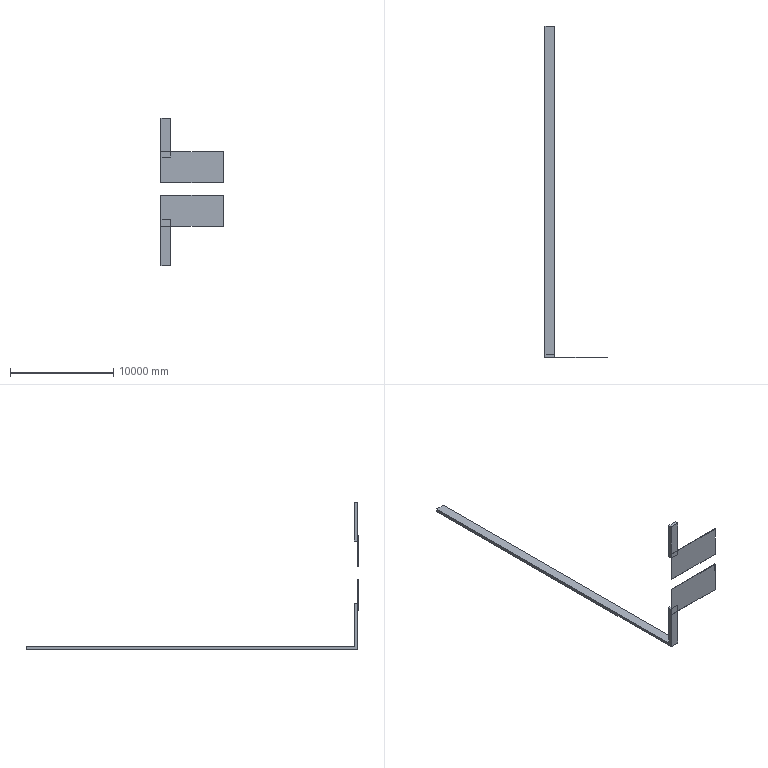Component | SolidWorks | Wall-1 | 4 solids | 26 faces | box 6000 x 32121.42 x 14227.61 mm | volume 12599737425 mm3 | plane 26
build123d program:
from build123d import *

# Parameters (mm, degrees)
BOSS_EXTRUDE1_DEPTH   = 900
SKETCH2_W             = 1916.372
SKETCH2_H             = 6000
CUT_EXTRUDE2_DEPTH    = 38704.356
SKETCH3_W             = 6000
SKETCH3_H             = 3000
BOSS_EXTRUDE2_DEPTH   = 50
BOSS_EXTRUDE2_2_DEPTH = 50


with BuildPart() as part:
    # Sketch1 → Boss-Extrude1 (new body)
    with BuildSketch(Plane.XY):
        Polygon((-3905.572, 13.034), (-35976.99, 13.034), (-35976.99, 313.034), (-35976.99, 14240.643), (-35676.99, 14240.643), (-35676.99, 313.034), (-3905.572, 313.034), align=None)
    extrude(amount=BOSS_EXTRUDE1_DEPTH)

    # Sketch2 → Cut-Extrude2 (cut, through all)
    with BuildSketch(Plane.XY.offset(900)):
        with Locations((-36116.386, 7513.034)):
            Rectangle(SKETCH2_W, SKETCH2_H)
    extrude(amount=-CUT_EXTRUDE2_DEPTH, mode=Mode.SUBTRACT)


with BuildPart() as cut_extrude2_piece_1:
    # of the separate pieces the step leaves, piece 1, a body of its own (cut_extrude2_pieces)
    add(part.part.solids().sort_by_distance((-3905.572, 13.034, 0))[0])


with BuildPart() as cut_extrude2_piece_2:
    # of the separate pieces the step leaves, piece 2, a body of its own (cut_extrude2_pieces)
    add(part.part.solids().sort_by_distance((-35976.99, 14240.643, 0))[0])


with BuildPart() as body_3:
    # Sketch3 → Boss-Extrude2 (new body)
    with BuildSketch(Plane.ZY.offset(35976.99)):
        with Locations((3000, 9513.138)):
            Rectangle(SKETCH3_W, SKETCH3_H)
    extrude(amount=BOSS_EXTRUDE2_DEPTH)


with BuildPart() as body_4:
    # Sketch3 → Boss-Extrude2 2 (new body)
    with BuildSketch(Plane.ZY.offset(35976.99)):
        with Locations((3000, 5329.239)):
            Rectangle(SKETCH3_W, SKETCH3_H)
    extrude(amount=BOSS_EXTRUDE2_2_DEPTH)


solid = Compound([cut_extrude2_piece_1.part, cut_extrude2_piece_2.part, body_3.part, body_4.part])

# Placed as in the assembly
solid = solid.moved(Location((-1730.074, 4663.226, -160.714), (90, 90, 0)))
STEP:
#1=CARTESIAN_POINT('',(-68.113,-1232.825,427.261));
#2=VERTEX_POINT('',#1);
#3=CARTESIAN_POINT('',(-68.113,-1232.825,309.151));
#4=VERTEX_POINT('',#3);
#5=CARTESIAN_POINT('',(-68.113,-1232.825,427.261));
#6=DIRECTION('',(-0.,-0.,-1.));
#7=VECTOR('',#6,39.37);
#8=LINE('',#5,#7);
#9=EDGE_CURVE('',#2,#4,#8,.T.);
#10=ORIENTED_EDGE('',*,*,#9,.T.);
#11=CARTESIAN_POINT('',(-68.113,-1234.794,309.151));
#12=VERTEX_POINT('',#11);
#13=CARTESIAN_POINT('',(-68.113,-1234.794,309.151));
#14=DIRECTION('',(0.,1.,-0.));
#15=VECTOR('',#14,39.37);
#16=LINE('',#13,#15);
#17=EDGE_CURVE('',#12,#4,#16,.T.);
#18=ORIENTED_EDGE('',*,*,#17,.F.);
#19=CARTESIAN_POINT('',(-68.113,-1234.794,427.261));
#20=VERTEX_POINT('',#19);
#21=CARTESIAN_POINT('',(-68.113,-1234.794,427.261));
#22=DIRECTION('',(-0.,-0.,-1.));
#23=VECTOR('',#22,39.37);
#24=LINE('',#21,#23);
#25=EDGE_CURVE('',#20,#12,#24,.T.);
#26=ORIENTED_EDGE('',*,*,#25,.F.);
#27=CARTESIAN_POINT('',(-68.113,-1234.794,427.261));
#28=DIRECTION('',(0.,1.,-0.));
#29=VECTOR('',#28,39.37);
#30=LINE('',#27,#29);
#31=EDGE_CURVE('',#20,#2,#30,.T.);
#32=ORIENTED_EDGE('',*,*,#31,.T.);
#33=EDGE_LOOP('',(#10,#18,#26,#32));
#34=FACE_OUTER_BOUND('',#33,.T.);
#35=CARTESIAN_POINT('',(-68.113,-1234.794,427.261));
#36=DIRECTION('',(1.,-0.,-0.));
#37=DIRECTION('',(-0.,-0.,-1.));
#38=AXIS2_PLACEMENT_3D('',#35,#36,#37);
#39=PLANE('',#38);
#40=ADVANCED_FACE('',(#34),#39,.F.);
#41=CARTESIAN_POINT('',(168.107,-1232.825,309.151));
#42=VERTEX_POINT('',#41);
#43=CARTESIAN_POINT('',(-68.113,-1232.825,309.151));
#44=DIRECTION('',(1.,-0.,-0.));
#45=VECTOR('',#44,39.37);
#46=LINE('',#43,#45);
#47=EDGE_CURVE('',#4,#42,#46,.T.);
#48=ORIENTED_EDGE('',*,*,#47,.T.);
#49=CARTESIAN_POINT('',(168.107,-1234.794,309.151));
#50=VERTEX_POINT('',#49);
#51=CARTESIAN_POINT('',(168.107,-1234.794,309.151));
#52=DIRECTION('',(0.,1.,-0.));
#53=VECTOR('',#52,39.37);
#54=LINE('',#51,#53);
#55=EDGE_CURVE('',#50,#42,#54,.T.);
#56=ORIENTED_EDGE('',*,*,#55,.F.);
#57=CARTESIAN_POINT('',(-68.113,-1234.794,309.151));
#58=DIRECTION('',(1.,-0.,-0.));
#59=VECTOR('',#58,39.37);
#60=LINE('',#57,#59);
#61=EDGE_CURVE('',#12,#50,#60,.T.);
#62=ORIENTED_EDGE('',*,*,#61,.F.);
#63=ORIENTED_EDGE('',*,*,#17,.T.);
#64=EDGE_LOOP('',(#48,#56,#62,#63));
#65=FACE_OUTER_BOUND('',#64,.T.);
#66=CARTESIAN_POINT('',(-68.113,-1234.794,309.151));
#67=DIRECTION('',(0.,0.,1.));
#68=DIRECTION('',(1.,-0.,-0.));
#69=AXIS2_PLACEMENT_3D('',#66,#67,#68);
#70=PLANE('',#69);
#71=ADVANCED_FACE('',(#65),#70,.F.);
#72=CARTESIAN_POINT('',(168.107,-1232.825,427.261));
#73=VERTEX_POINT('',#72);
#74=CARTESIAN_POINT('',(168.107,-1232.825,427.261));
#75=DIRECTION('',(0.,0.,1.));
#76=VECTOR('',#75,39.37);
#77=LINE('',#74,#76);
#78=EDGE_CURVE('',#42,#73,#77,.T.);
#79=ORIENTED_EDGE('',*,*,#78,.T.);
#80=CARTESIAN_POINT('',(168.107,-1234.794,427.261));
#81=VERTEX_POINT('',#80);
#82=CARTESIAN_POINT('',(168.107,-1234.794,427.261));
#83=DIRECTION('',(0.,1.,-0.));
#84=VECTOR('',#83,39.37);
#85=LINE('',#82,#84);
#86=EDGE_CURVE('',#81,#73,#85,.T.);
#87=ORIENTED_EDGE('',*,*,#86,.F.);
#88=CARTESIAN_POINT('',(168.107,-1234.794,427.261));
#89=DIRECTION('',(0.,0.,1.));
#90=VECTOR('',#89,39.37);
#91=LINE('',#88,#90);
#92=EDGE_CURVE('',#50,#81,#91,.T.);
#93=ORIENTED_EDGE('',*,*,#92,.F.);
#94=ORIENTED_EDGE('',*,*,#55,.T.);
#95=EDGE_LOOP('',(#79,#87,#93,#94));
#96=FACE_OUTER_BOUND('',#95,.T.);
#97=CARTESIAN_POINT('',(168.107,-1234.794,427.261));
#98=DIRECTION('',(-1.,0.,0.));
#99=DIRECTION('',(-0.,-1.,0.));
#100=AXIS2_PLACEMENT_3D('',#97,#98,#99);
#101=PLANE('',#100);
#102=ADVANCED_FACE('',(#96),#101,.F.);
#103=CARTESIAN_POINT('',(-68.113,-1232.825,427.261));
#104=DIRECTION('',(-1.,0.,0.));
#105=VECTOR('',#104,39.37);
#106=LINE('',#103,#105);
#107=EDGE_CURVE('',#73,#2,#106,.T.);
#108=ORIENTED_EDGE('',*,*,#107,.T.);
#109=ORIENTED_EDGE('',*,*,#31,.F.);
#110=CARTESIAN_POINT('',(-68.113,-1234.794,427.261));
#111=DIRECTION('',(-1.,0.,0.));
#112=VECTOR('',#111,39.37);
#113=LINE('',#110,#112);
#114=EDGE_CURVE('',#81,#20,#113,.T.);
#115=ORIENTED_EDGE('',*,*,#114,.F.);
#116=ORIENTED_EDGE('',*,*,#86,.T.);
#117=EDGE_LOOP('',(#108,#109,#115,#116));
#118=FACE_OUTER_BOUND('',#117,.T.);
#119=CARTESIAN_POINT('',(-68.113,-1234.794,427.261));
#120=DIRECTION('',(-0.,-0.,-1.));
#121=DIRECTION('',(-1.,0.,0.));
#122=AXIS2_PLACEMENT_3D('',#119,#120,#121);
#123=PLANE('',#122);
#124=ADVANCED_FACE('',(#118),#123,.F.);
#125=ORIENTED_EDGE('',*,*,#25,.T.);
#126=ORIENTED_EDGE('',*,*,#61,.T.);
#127=ORIENTED_EDGE('',*,*,#92,.T.);
#128=ORIENTED_EDGE('',*,*,#114,.T.);
#129=EDGE_LOOP('',(#125,#126,#127,#128));
#130=FACE_OUTER_BOUND('',#129,.T.);
#131=CARTESIAN_POINT('',(-68.113,-1234.794,-6.327));
#132=DIRECTION('',(-0.,-1.,0.));
#133=DIRECTION('',(1.,-0.,-0.));
#134=AXIS2_PLACEMENT_3D('',#131,#132,#133);
#135=PLANE('',#134);
#136=ADVANCED_FACE('',(#130),#135,.T.);
#137=ORIENTED_EDGE('',*,*,#9,.F.);
#138=ORIENTED_EDGE('',*,*,#107,.F.);
#139=ORIENTED_EDGE('',*,*,#78,.F.);
#140=ORIENTED_EDGE('',*,*,#47,.F.);
#141=EDGE_LOOP('',(#137,#138,#139,#140));
#142=FACE_OUTER_BOUND('',#141,.T.);
#143=CARTESIAN_POINT('',(-68.113,-1232.825,-6.327));
#144=DIRECTION('',(-0.,-1.,0.));
#145=DIRECTION('',(1.,-0.,-0.));
#146=AXIS2_PLACEMENT_3D('',#143,#144,#145);
#147=PLANE('',#146);
#148=ADVANCED_FACE('',(#142),#147,.F.);
#149=CLOSED_SHELL('',(#40,#71,#102,#124,#136,#148));
#150=MANIFOLD_SOLID_BREP('',#149);
#151=CARTESIAN_POINT('',(-68.113,-1232.825,554.328));
#152=VERTEX_POINT('',#151);
#153=CARTESIAN_POINT('',(-68.113,-1221.014,554.328));
#154=VERTEX_POINT('',#153);
#155=CARTESIAN_POINT('',(-68.113,-1232.825,554.328));
#156=DIRECTION('',(0.,1.,-0.));
#157=VECTOR('',#156,39.37);
#158=LINE('',#155,#157);
#159=EDGE_CURVE('',#152,#154,#158,.T.);
#160=ORIENTED_EDGE('',*,*,#159,.F.);
#161=CARTESIAN_POINT('',(-32.68,-1232.825,554.328));
#162=VERTEX_POINT('',#161);
#163=CARTESIAN_POINT('',(-32.68,-1232.825,554.328));
#164=DIRECTION('',(-1.,0.,0.));
#165=VECTOR('',#164,39.37);
#166=LINE('',#163,#165);
#167=EDGE_CURVE('',#162,#152,#166,.T.);
#168=ORIENTED_EDGE('',*,*,#167,.F.);
#169=CARTESIAN_POINT('',(-32.68,-1221.014,554.328));
#170=VERTEX_POINT('',#169);
#171=CARTESIAN_POINT('',(-32.68,-1232.825,554.328));
#172=DIRECTION('',(0.,1.,-0.));
#173=VECTOR('',#172,39.37);
#174=LINE('',#171,#173);
#175=EDGE_CURVE('',#162,#170,#174,.T.);
#176=ORIENTED_EDGE('',*,*,#175,.T.);
#177=CARTESIAN_POINT('',(-32.68,-1221.014,554.328));
#178=DIRECTION('',(-1.,0.,0.));
#179=VECTOR('',#178,39.37);
#180=LINE('',#177,#179);
#181=EDGE_CURVE('',#170,#154,#180,.T.);
#182=ORIENTED_EDGE('',*,*,#181,.T.);
#183=EDGE_LOOP('',(#160,#168,#176,#182));
#184=FACE_OUTER_BOUND('',#183,.T.);
#185=CARTESIAN_POINT('',(-32.68,-1232.825,554.328));
#186=DIRECTION('',(0.,0.,1.));
#187=DIRECTION('',(1.,-0.,-0.));
#188=AXIS2_PLACEMENT_3D('',#185,#186,#187);
#189=PLANE('',#188);
#190=ADVANCED_FACE('',(#184),#189,.T.);
#191=CARTESIAN_POINT('',(-68.113,-1232.825,407.572));
#192=VERTEX_POINT('',#191);
#193=CARTESIAN_POINT('',(-68.113,-1221.014,407.572));
#194=VERTEX_POINT('',#193);
#195=CARTESIAN_POINT('',(-68.113,183.592,407.572));
#196=DIRECTION('',(0.,1.,-0.));
#197=VECTOR('',#196,39.37);
#198=LINE('',#195,#197);
#199=EDGE_CURVE('',#192,#194,#198,.T.);
#200=ORIENTED_EDGE('',*,*,#199,.F.);
#201=CARTESIAN_POINT('',(-68.113,-1232.825,5.997));
#202=DIRECTION('',(0.,0.,1.));
#203=VECTOR('',#202,39.37);
#204=LINE('',#201,#203);
#205=EDGE_CURVE('',#192,#152,#204,.T.);
#206=ORIENTED_EDGE('',*,*,#205,.T.);
#207=ORIENTED_EDGE('',*,*,#159,.T.);
#208=CARTESIAN_POINT('',(-68.113,-1221.014,5.997));
#209=DIRECTION('',(0.,0.,1.));
#210=VECTOR('',#209,39.37);
#211=LINE('',#208,#210);
#212=EDGE_CURVE('',#194,#154,#211,.T.);
#213=ORIENTED_EDGE('',*,*,#212,.F.);
#214=EDGE_LOOP('',(#200,#206,#207,#213));
#215=FACE_OUTER_BOUND('',#214,.T.);
#216=CARTESIAN_POINT('',(-68.113,183.592,-6.327));
#217=DIRECTION('',(-1.,0.,0.));
#218=DIRECTION('',(-0.,-1.,0.));
#219=AXIS2_PLACEMENT_3D('',#216,#217,#218);
#220=PLANE('',#219);
#221=ADVANCED_FACE('',(#215),#220,.T.);
#222=CARTESIAN_POINT('',(-32.68,-1232.825,407.572));
#223=VERTEX_POINT('',#222);
#224=CARTESIAN_POINT('',(-32.68,-1232.825,-5.814));
#225=DIRECTION('',(0.,0.,1.));
#226=VECTOR('',#225,39.37);
#227=LINE('',#224,#226);
#228=EDGE_CURVE('',#223,#162,#227,.T.);
#229=ORIENTED_EDGE('',*,*,#228,.F.);
#230=CARTESIAN_POINT('',(-32.68,-1221.014,407.572));
#231=VERTEX_POINT('',#230);
#232=CARTESIAN_POINT('',(-32.68,-1200.59,407.572));
#233=DIRECTION('',(-0.,-1.,0.));
#234=VECTOR('',#233,39.37);
#235=LINE('',#232,#234);
#236=EDGE_CURVE('',#231,#223,#235,.T.);
#237=ORIENTED_EDGE('',*,*,#236,.F.);
#238=CARTESIAN_POINT('',(-32.68,-1221.014,5.997));
#239=DIRECTION('',(0.,0.,1.));
#240=VECTOR('',#239,39.37);
#241=LINE('',#238,#240);
#242=EDGE_CURVE('',#231,#170,#241,.T.);
#243=ORIENTED_EDGE('',*,*,#242,.T.);
#244=ORIENTED_EDGE('',*,*,#175,.F.);
#245=EDGE_LOOP('',(#229,#237,#243,#244));
#246=FACE_OUTER_BOUND('',#245,.T.);
#247=CARTESIAN_POINT('',(-32.68,183.592,-6.327));
#248=DIRECTION('',(-1.,0.,0.));
#249=DIRECTION('',(-0.,-1.,0.));
#250=AXIS2_PLACEMENT_3D('',#247,#248,#249);
#251=PLANE('',#250);
#252=ADVANCED_FACE('',(#246),#251,.F.);
#253=CARTESIAN_POINT('',(-32.68,-1232.825,407.572));
#254=DIRECTION('',(-1.,0.,0.));
#255=VECTOR('',#254,39.37);
#256=LINE('',#253,#255);
#257=EDGE_CURVE('',#223,#192,#256,.T.);
#258=ORIENTED_EDGE('',*,*,#257,.F.);
#259=ORIENTED_EDGE('',*,*,#228,.T.);
#260=ORIENTED_EDGE('',*,*,#167,.T.);
#261=ORIENTED_EDGE('',*,*,#205,.F.);
#262=EDGE_LOOP('',(#258,#259,#260,#261));
#263=FACE_OUTER_BOUND('',#262,.T.);
#264=CARTESIAN_POINT('',(-32.68,-1232.825,5.997));
#265=DIRECTION('',(-0.,-1.,0.));
#266=DIRECTION('',(1.,-0.,-0.));
#267=AXIS2_PLACEMENT_3D('',#264,#265,#266);
#268=PLANE('',#267);
#269=ADVANCED_FACE('',(#263),#268,.T.);
#270=ORIENTED_EDGE('',*,*,#242,.F.);
#271=CARTESIAN_POINT('',(-32.68,-1221.014,407.572));
#272=DIRECTION('',(-1.,0.,0.));
#273=VECTOR('',#272,39.37);
#274=LINE('',#271,#273);
#275=EDGE_CURVE('',#231,#194,#274,.T.);
#276=ORIENTED_EDGE('',*,*,#275,.T.);
#277=ORIENTED_EDGE('',*,*,#212,.T.);
#278=ORIENTED_EDGE('',*,*,#181,.F.);
#279=EDGE_LOOP('',(#270,#276,#277,#278));
#280=FACE_OUTER_BOUND('',#279,.T.);
#281=CARTESIAN_POINT('',(-32.68,-1221.014,5.997));
#282=DIRECTION('',(-0.,-1.,0.));
#283=DIRECTION('',(1.,-0.,-0.));
#284=AXIS2_PLACEMENT_3D('',#281,#282,#283);
#285=PLANE('',#284);
#286=ADVANCED_FACE('',(#280),#285,.F.);
#287=ORIENTED_EDGE('',*,*,#236,.T.);
#288=ORIENTED_EDGE('',*,*,#257,.T.);
#289=ORIENTED_EDGE('',*,*,#199,.T.);
#290=ORIENTED_EDGE('',*,*,#275,.F.);
#291=EDGE_LOOP('',(#287,#288,#289,#290));
#292=FACE_OUTER_BOUND('',#291,.T.);
#293=CARTESIAN_POINT('',(-68.113,-1200.59,407.572));
#294=DIRECTION('',(0.,0.,1.));
#295=DIRECTION('',(1.,-0.,-0.));
#296=AXIS2_PLACEMENT_3D('',#293,#294,#295);
#297=PLANE('',#296);
#298=ADVANCED_FACE('',(#292),#297,.F.);
#299=CLOSED_SHELL('',(#190,#221,#252,#269,#286,#298));
#300=MANIFOLD_SOLID_BREP('',#299);
#301=CARTESIAN_POINT('',(-68.113,-1221.014,5.997));
#302=VERTEX_POINT('',#301);
#303=CARTESIAN_POINT('',(-68.113,-1221.014,171.351));
#304=VERTEX_POINT('',#303);
#305=CARTESIAN_POINT('',(-68.113,-1221.014,5.997));
#306=DIRECTION('',(0.,0.,1.));
#307=VECTOR('',#306,39.37);
#308=LINE('',#305,#307);
#309=EDGE_CURVE('',#302,#304,#308,.T.);
#310=ORIENTED_EDGE('',*,*,#309,.T.);
#311=CARTESIAN_POINT('',(-32.68,-1221.014,171.351));
#312=VERTEX_POINT('',#311);
#313=CARTESIAN_POINT('',(-32.68,-1221.014,171.351));
#314=DIRECTION('',(1.,-0.,-0.));
#315=VECTOR('',#314,39.37);
#316=LINE('',#313,#315);
#317=EDGE_CURVE('',#304,#312,#316,.T.);
#318=ORIENTED_EDGE('',*,*,#317,.T.);
#319=CARTESIAN_POINT('',(-32.68,-1221.014,5.997));
#320=VERTEX_POINT('',#319);
#321=CARTESIAN_POINT('',(-32.68,-1221.014,5.997));
#322=DIRECTION('',(0.,0.,1.));
#323=VECTOR('',#322,39.37);
#324=LINE('',#321,#323);
#325=EDGE_CURVE('',#320,#312,#324,.T.);
#326=ORIENTED_EDGE('',*,*,#325,.F.);
#327=CARTESIAN_POINT('',(-32.68,-1221.014,5.997));
#328=DIRECTION('',(-1.,0.,0.));
#329=VECTOR('',#328,39.37);
#330=LINE('',#327,#329);
#331=EDGE_CURVE('',#320,#302,#330,.T.);
#332=ORIENTED_EDGE('',*,*,#331,.T.);
#333=EDGE_LOOP('',(#310,#318,#326,#332));
#334=FACE_OUTER_BOUND('',#333,.T.);
#335=CARTESIAN_POINT('',(-32.68,-1221.014,5.997));
#336=DIRECTION('',(-0.,-1.,0.));
#337=DIRECTION('',(1.,-0.,-0.));
#338=AXIS2_PLACEMENT_3D('',#335,#336,#337);
#339=PLANE('',#338);
#340=ADVANCED_FACE('',(#334),#339,.F.);
#341=CARTESIAN_POINT('',(-68.113,-1232.825,171.351));
#342=VERTEX_POINT('',#341);
#343=CARTESIAN_POINT('',(-32.68,-1232.825,171.351));
#344=VERTEX_POINT('',#343);
#345=CARTESIAN_POINT('',(-32.68,-1232.825,171.351));
#346=DIRECTION('',(1.,-0.,-0.));
#347=VECTOR('',#346,39.37);
#348=LINE('',#345,#347);
#349=EDGE_CURVE('',#342,#344,#348,.T.);
#350=ORIENTED_EDGE('',*,*,#349,.F.);
#351=CARTESIAN_POINT('',(-68.113,-1232.825,-5.814));
#352=VERTEX_POINT('',#351);
#353=CARTESIAN_POINT('',(-68.113,-1232.825,5.997));
#354=DIRECTION('',(0.,0.,1.));
#355=VECTOR('',#354,39.37);
#356=LINE('',#353,#355);
#357=EDGE_CURVE('',#352,#342,#356,.T.);
#358=ORIENTED_EDGE('',*,*,#357,.F.);
#359=CARTESIAN_POINT('',(-32.68,-1232.825,-5.814));
#360=VERTEX_POINT('',#359);
#361=CARTESIAN_POINT('',(-32.68,-1232.825,-5.814));
#362=DIRECTION('',(-1.,0.,0.));
#363=VECTOR('',#362,39.37);
#364=LINE('',#361,#363);
#365=EDGE_CURVE('',#360,#352,#364,.T.);
#366=ORIENTED_EDGE('',*,*,#365,.F.);
#367=CARTESIAN_POINT('',(-32.68,-1232.825,-5.814));
#368=DIRECTION('',(0.,0.,1.));
#369=VECTOR('',#368,39.37);
#370=LINE('',#367,#369);
#371=EDGE_CURVE('',#360,#344,#370,.T.);
#372=ORIENTED_EDGE('',*,*,#371,.T.);
#373=EDGE_LOOP('',(#350,#358,#366,#372));
#374=FACE_OUTER_BOUND('',#373,.T.);
#375=CARTESIAN_POINT('',(-32.68,-1232.825,5.997));
#376=DIRECTION('',(-0.,-1.,0.));
#377=DIRECTION('',(1.,-0.,-0.));
#378=AXIS2_PLACEMENT_3D('',#375,#376,#377);
#379=PLANE('',#378);
#380=ADVANCED_FACE('',(#374),#379,.T.);
#381=ORIENTED_EDGE('',*,*,#325,.T.);
#382=CARTESIAN_POINT('',(-32.68,-1200.59,171.351));
#383=DIRECTION('',(0.,1.,-0.));
#384=VECTOR('',#383,39.37);
#385=LINE('',#382,#384);
#386=EDGE_CURVE('',#344,#312,#385,.T.);
#387=ORIENTED_EDGE('',*,*,#386,.F.);
#388=ORIENTED_EDGE('',*,*,#371,.F.);
#389=CARTESIAN_POINT('',(-32.68,29.829,-5.814));
#390=VERTEX_POINT('',#389);
#391=CARTESIAN_POINT('',(-32.68,29.829,-5.814));
#392=DIRECTION('',(-0.,-1.,0.));
#393=VECTOR('',#392,39.37);
#394=LINE('',#391,#393);
#395=EDGE_CURVE('',#390,#360,#394,.T.);
#396=ORIENTED_EDGE('',*,*,#395,.F.);
#397=CARTESIAN_POINT('',(-32.68,29.829,5.997));
#398=VERTEX_POINT('',#397);
#399=CARTESIAN_POINT('',(-32.68,29.829,-5.814));
#400=DIRECTION('',(0.,0.,1.));
#401=VECTOR('',#400,39.37);
#402=LINE('',#399,#401);
#403=EDGE_CURVE('',#390,#398,#402,.T.);
#404=ORIENTED_EDGE('',*,*,#403,.T.);
#405=CARTESIAN_POINT('',(-32.68,29.829,5.997));
#406=DIRECTION('',(-0.,-1.,0.));
#407=VECTOR('',#406,39.37);
#408=LINE('',#405,#407);
#409=EDGE_CURVE('',#398,#320,#408,.T.);
#410=ORIENTED_EDGE('',*,*,#409,.T.);
#411=EDGE_LOOP('',(#381,#387,#388,#396,#404,#410));
#412=FACE_OUTER_BOUND('',#411,.T.);
#413=CARTESIAN_POINT('',(-32.68,183.592,-6.327));
#414=DIRECTION('',(-1.,0.,0.));
#415=DIRECTION('',(-0.,-1.,0.));
#416=AXIS2_PLACEMENT_3D('',#413,#414,#415);
#417=PLANE('',#416);
#418=ADVANCED_FACE('',(#412),#417,.F.);
#419=CARTESIAN_POINT('',(-68.113,183.592,171.351));
#420=DIRECTION('',(-0.,-1.,0.));
#421=VECTOR('',#420,39.37);
#422=LINE('',#419,#421);
#423=EDGE_CURVE('',#304,#342,#422,.T.);
#424=ORIENTED_EDGE('',*,*,#423,.F.);
#425=ORIENTED_EDGE('',*,*,#309,.F.);
#426=CARTESIAN_POINT('',(-68.113,29.829,5.997));
#427=VERTEX_POINT('',#426);
#428=CARTESIAN_POINT('',(-68.113,29.829,5.997));
#429=DIRECTION('',(-0.,-1.,0.));
#430=VECTOR('',#429,39.37);
#431=LINE('',#428,#430);
#432=EDGE_CURVE('',#427,#302,#431,.T.);
#433=ORIENTED_EDGE('',*,*,#432,.F.);
#434=CARTESIAN_POINT('',(-68.113,29.829,-5.814));
#435=VERTEX_POINT('',#434);
#436=CARTESIAN_POINT('',(-68.113,29.829,-5.814));
#437=DIRECTION('',(0.,0.,1.));
#438=VECTOR('',#437,39.37);
#439=LINE('',#436,#438);
#440=EDGE_CURVE('',#435,#427,#439,.T.);
#441=ORIENTED_EDGE('',*,*,#440,.F.);
#442=CARTESIAN_POINT('',(-68.113,29.829,-5.814));
#443=DIRECTION('',(-0.,-1.,0.));
#444=VECTOR('',#443,39.37);
#445=LINE('',#442,#444);
#446=EDGE_CURVE('',#435,#352,#445,.T.);
#447=ORIENTED_EDGE('',*,*,#446,.T.);
#448=ORIENTED_EDGE('',*,*,#357,.T.);
#449=EDGE_LOOP('',(#424,#425,#433,#441,#447,#448));
#450=FACE_OUTER_BOUND('',#449,.T.);
#451=CARTESIAN_POINT('',(-68.113,183.592,-6.327));
#452=DIRECTION('',(-1.,0.,0.));
#453=DIRECTION('',(-0.,-1.,0.));
#454=AXIS2_PLACEMENT_3D('',#451,#452,#453);
#455=PLANE('',#454);
#456=ADVANCED_FACE('',(#450),#455,.T.);
#457=ORIENTED_EDGE('',*,*,#446,.F.);
#458=CARTESIAN_POINT('',(-32.68,29.829,-5.814));
#459=DIRECTION('',(-1.,0.,0.));
#460=VECTOR('',#459,39.37);
#461=LINE('',#458,#460);
#462=EDGE_CURVE('',#390,#435,#461,.T.);
#463=ORIENTED_EDGE('',*,*,#462,.F.);
#464=ORIENTED_EDGE('',*,*,#395,.T.);
#465=ORIENTED_EDGE('',*,*,#365,.T.);
#466=EDGE_LOOP('',(#457,#463,#464,#465));
#467=FACE_OUTER_BOUND('',#466,.T.);
#468=CARTESIAN_POINT('',(-32.68,29.829,-5.814));
#469=DIRECTION('',(-0.,-0.,-1.));
#470=DIRECTION('',(-1.,0.,0.));
#471=AXIS2_PLACEMENT_3D('',#468,#469,#470);
#472=PLANE('',#471);
#473=ADVANCED_FACE('',(#467),#472,.T.);
#474=ORIENTED_EDGE('',*,*,#440,.T.);
#475=CARTESIAN_POINT('',(-32.68,29.829,5.997));
#476=DIRECTION('',(-1.,0.,0.));
#477=VECTOR('',#476,39.37);
#478=LINE('',#475,#477);
#479=EDGE_CURVE('',#398,#427,#478,.T.);
#480=ORIENTED_EDGE('',*,*,#479,.F.);
#481=ORIENTED_EDGE('',*,*,#403,.F.);
#482=ORIENTED_EDGE('',*,*,#462,.T.);
#483=EDGE_LOOP('',(#474,#480,#481,#482));
#484=FACE_OUTER_BOUND('',#483,.T.);
#485=CARTESIAN_POINT('',(-32.68,29.829,-5.814));
#486=DIRECTION('',(-0.,-1.,0.));
#487=DIRECTION('',(1.,-0.,-0.));
#488=AXIS2_PLACEMENT_3D('',#485,#486,#487);
#489=PLANE('',#488);
#490=ADVANCED_FACE('',(#484),#489,.F.);
#491=ORIENTED_EDGE('',*,*,#432,.T.);
#492=ORIENTED_EDGE('',*,*,#331,.F.);
#493=ORIENTED_EDGE('',*,*,#409,.F.);
#494=ORIENTED_EDGE('',*,*,#479,.T.);
#495=EDGE_LOOP('',(#491,#492,#493,#494));
#496=FACE_OUTER_BOUND('',#495,.T.);
#497=CARTESIAN_POINT('',(-32.68,29.829,5.997));
#498=DIRECTION('',(-0.,-0.,-1.));
#499=DIRECTION('',(-1.,0.,0.));
#500=AXIS2_PLACEMENT_3D('',#497,#498,#499);
#501=PLANE('',#500);
#502=ADVANCED_FACE('',(#496),#501,.F.);
#503=ORIENTED_EDGE('',*,*,#423,.T.);
#504=ORIENTED_EDGE('',*,*,#349,.T.);
#505=ORIENTED_EDGE('',*,*,#386,.T.);
#506=ORIENTED_EDGE('',*,*,#317,.F.);
#507=EDGE_LOOP('',(#503,#504,#505,#506));
#508=FACE_OUTER_BOUND('',#507,.T.);
#509=CARTESIAN_POINT('',(-68.113,-1200.59,171.351));
#510=DIRECTION('',(-0.,-0.,-1.));
#511=DIRECTION('',(-1.,0.,0.));
#512=AXIS2_PLACEMENT_3D('',#509,#510,#511);
#513=PLANE('',#512);
#514=ADVANCED_FACE('',(#508),#513,.F.);
#515=CLOSED_SHELL('',(#340,#380,#418,#456,#473,#490,#502,#514));
#516=MANIFOLD_SOLID_BREP('',#515);
#517=CARTESIAN_POINT('',(-68.113,-1232.825,262.54));
#518=VERTEX_POINT('',#517);
#519=CARTESIAN_POINT('',(-68.113,-1232.825,144.43));
#520=VERTEX_POINT('',#519);
#521=CARTESIAN_POINT('',(-68.113,-1232.825,144.43));
#522=DIRECTION('',(-0.,-0.,-1.));
#523=VECTOR('',#522,39.37);
#524=LINE('',#521,#523);
#525=EDGE_CURVE('',#518,#520,#524,.T.);
#526=ORIENTED_EDGE('',*,*,#525,.T.);
#527=CARTESIAN_POINT('',(-68.113,-1234.794,144.43));
#528=VERTEX_POINT('',#527);
#529=CARTESIAN_POINT('',(-68.113,-1234.794,144.43));
#530=DIRECTION('',(0.,1.,-0.));
#531=VECTOR('',#530,39.37);
#532=LINE('',#529,#531);
#533=EDGE_CURVE('',#528,#520,#532,.T.);
#534=ORIENTED_EDGE('',*,*,#533,.F.);
#535=CARTESIAN_POINT('',(-68.113,-1234.794,262.54));
#536=VERTEX_POINT('',#535);
#537=CARTESIAN_POINT('',(-68.113,-1234.794,144.43));
#538=DIRECTION('',(-0.,-0.,-1.));
#539=VECTOR('',#538,39.37);
#540=LINE('',#537,#539);
#541=EDGE_CURVE('',#536,#528,#540,.T.);
#542=ORIENTED_EDGE('',*,*,#541,.F.);
#543=CARTESIAN_POINT('',(-68.113,-1234.794,262.54));
#544=DIRECTION('',(0.,1.,-0.));
#545=VECTOR('',#544,39.37);
#546=LINE('',#543,#545);
#547=EDGE_CURVE('',#536,#518,#546,.T.);
#548=ORIENTED_EDGE('',*,*,#547,.T.);
#549=EDGE_LOOP('',(#526,#534,#542,#548));
#550=FACE_OUTER_BOUND('',#549,.T.);
#551=CARTESIAN_POINT('',(-68.113,-1234.794,144.43));
#552=DIRECTION('',(1.,-0.,-0.));
#553=DIRECTION('',(0.,1.,-0.));
#554=AXIS2_PLACEMENT_3D('',#551,#552,#553);
#555=PLANE('',#554);
#556=ADVANCED_FACE('',(#550),#555,.F.);
#557=CARTESIAN_POINT('',(168.107,-1232.825,144.43));
#558=VERTEX_POINT('',#557);
#559=CARTESIAN_POINT('',(-68.113,-1232.825,144.43));
#560=DIRECTION('',(1.,-0.,-0.));
#561=VECTOR('',#560,39.37);
#562=LINE('',#559,#561);
#563=EDGE_CURVE('',#520,#558,#562,.T.);
#564=ORIENTED_EDGE('',*,*,#563,.T.);
#565=CARTESIAN_POINT('',(168.107,-1234.794,144.43));
#566=VERTEX_POINT('',#565);
#567=CARTESIAN_POINT('',(168.107,-1234.794,144.43));
#568=DIRECTION('',(0.,1.,-0.));
#569=VECTOR('',#568,39.37);
#570=LINE('',#567,#569);
#571=EDGE_CURVE('',#566,#558,#570,.T.);
#572=ORIENTED_EDGE('',*,*,#571,.F.);
#573=CARTESIAN_POINT('',(-68.113,-1234.794,144.43));
#574=DIRECTION('',(1.,-0.,-0.));
#575=VECTOR('',#574,39.37);
#576=LINE('',#573,#575);
#577=EDGE_CURVE('',#528,#566,#576,.T.);
#578=ORIENTED_EDGE('',*,*,#577,.F.);
#579=ORIENTED_EDGE('',*,*,#533,.T.);
#580=EDGE_LOOP('',(#564,#572,#578,#579));
#581=FACE_OUTER_BOUND('',#580,.T.);
#582=CARTESIAN_POINT('',(-68.113,-1234.794,144.43));
#583=DIRECTION('',(0.,0.,1.));
#584=DIRECTION('',(1.,-0.,-0.));
#585=AXIS2_PLACEMENT_3D('',#582,#583,#584);
#586=PLANE('',#585);
#587=ADVANCED_FACE('',(#581),#586,.F.);
#588=CARTESIAN_POINT('',(168.107,-1232.825,262.54));
#589=VERTEX_POINT('',#588);
#590=CARTESIAN_POINT('',(168.107,-1232.825,144.43));
#591=DIRECTION('',(0.,0.,1.));
#592=VECTOR('',#591,39.37);
#593=LINE('',#590,#592);
#594=EDGE_CURVE('',#558,#589,#593,.T.);
#595=ORIENTED_EDGE('',*,*,#594,.T.);
#596=CARTESIAN_POINT('',(168.107,-1234.794,262.54));
#597=VERTEX_POINT('',#596);
#598=CARTESIAN_POINT('',(168.107,-1234.794,262.54));
#599=DIRECTION('',(0.,1.,-0.));
#600=VECTOR('',#599,39.37);
#601=LINE('',#598,#600);
#602=EDGE_CURVE('',#597,#589,#601,.T.);
#603=ORIENTED_EDGE('',*,*,#602,.F.);
#604=CARTESIAN_POINT('',(168.107,-1234.794,144.43));
#605=DIRECTION('',(0.,0.,1.));
#606=VECTOR('',#605,39.37);
#607=LINE('',#604,#606);
#608=EDGE_CURVE('',#566,#597,#607,.T.);
#609=ORIENTED_EDGE('',*,*,#608,.F.);
#610=ORIENTED_EDGE('',*,*,#571,.T.);
#611=EDGE_LOOP('',(#595,#603,#609,#610));
#612=FACE_OUTER_BOUND('',#611,.T.);
#613=CARTESIAN_POINT('',(168.107,-1234.794,144.43));
#614=DIRECTION('',(-1.,0.,0.));
#615=DIRECTION('',(-0.,-1.,0.));
#616=AXIS2_PLACEMENT_3D('',#613,#614,#615);
#617=PLANE('',#616);
#618=ADVANCED_FACE('',(#612),#617,.F.);
#619=CARTESIAN_POINT('',(-68.113,-1232.825,262.54));
#620=DIRECTION('',(-1.,0.,0.));
#621=VECTOR('',#620,39.37);
#622=LINE('',#619,#621);
#623=EDGE_CURVE('',#589,#518,#622,.T.);
#624=ORIENTED_EDGE('',*,*,#623,.T.);
#625=ORIENTED_EDGE('',*,*,#547,.F.);
#626=CARTESIAN_POINT('',(-68.113,-1234.794,262.54));
#627=DIRECTION('',(-1.,0.,0.));
#628=VECTOR('',#627,39.37);
#629=LINE('',#626,#628);
#630=EDGE_CURVE('',#597,#536,#629,.T.);
#631=ORIENTED_EDGE('',*,*,#630,.F.);
#632=ORIENTED_EDGE('',*,*,#602,.T.);
#633=EDGE_LOOP('',(#624,#625,#631,#632));
#634=FACE_OUTER_BOUND('',#633,.T.);
#635=CARTESIAN_POINT('',(-68.113,-1234.794,262.54));
#636=DIRECTION('',(-0.,-0.,-1.));
#637=DIRECTION('',(-1.,0.,0.));
#638=AXIS2_PLACEMENT_3D('',#635,#636,#637);
#639=PLANE('',#638);
#640=ADVANCED_FACE('',(#634),#639,.F.);
#641=ORIENTED_EDGE('',*,*,#541,.T.);
#642=ORIENTED_EDGE('',*,*,#577,.T.);
#643=ORIENTED_EDGE('',*,*,#608,.T.);
#644=ORIENTED_EDGE('',*,*,#630,.T.);
#645=EDGE_LOOP('',(#641,#642,#643,#644));
#646=FACE_OUTER_BOUND('',#645,.T.);
#647=CARTESIAN_POINT('',(-68.113,-1234.794,-6.327));
#648=DIRECTION('',(0.,1.,-0.));
#649=DIRECTION('',(-1.,0.,0.));
#650=AXIS2_PLACEMENT_3D('',#647,#648,#649);
#651=PLANE('',#650);
#652=ADVANCED_FACE('',(#646),#651,.F.);
#653=ORIENTED_EDGE('',*,*,#525,.F.);
#654=ORIENTED_EDGE('',*,*,#623,.F.);
#655=ORIENTED_EDGE('',*,*,#594,.F.);
#656=ORIENTED_EDGE('',*,*,#563,.F.);
#657=EDGE_LOOP('',(#653,#654,#655,#656));
#658=FACE_OUTER_BOUND('',#657,.T.);
#659=CARTESIAN_POINT('',(-68.113,-1232.825,-6.327));
#660=DIRECTION('',(0.,1.,-0.));
#661=DIRECTION('',(-1.,0.,0.));
#662=AXIS2_PLACEMENT_3D('',#659,#660,#661);
#663=PLANE('',#662);
#664=ADVANCED_FACE('',(#658),#663,.T.);
#665=CLOSED_SHELL('',(#556,#587,#618,#640,#652,#664));
#666=MANIFOLD_SOLID_BREP('',#665);
#667=CARTESIAN_POINT('',(0.,0.,0.));
#668=DIRECTION('',(0.,0.,1.));
#669=DIRECTION('',(1.,0.,0.));
#670=AXIS2_PLACEMENT_3D('',#667,#668,#669);
#671=(LENGTH_UNIT()NAMED_UNIT(*)SI_UNIT($,.METRE.));
#672=LENGTH_MEASURE_WITH_UNIT(LENGTH_MEASURE(0.0254),#671);
#673=DIMENSIONAL_EXPONENTS(1.,0.,0.,0.,0.,0.,0.);
#674=(CONVERSION_BASED_UNIT('',#672)LENGTH_UNIT()NAMED_UNIT(#673));
#675=UNCERTAINTY_MEASURE_WITH_UNIT(LENGTH_MEASURE(0.00001),#674,'','');
#676=(NAMED_UNIT(*)PLANE_ANGLE_UNIT()SI_UNIT($,.RADIAN.));
#677=(NAMED_UNIT(*)SI_UNIT($,.STERADIAN.)SOLID_ANGLE_UNIT());
#678=(GEOMETRIC_REPRESENTATION_CONTEXT(3)GLOBAL_UNCERTAINTY_ASSIGNED_CONTEXT((#675))GLOBAL_UNIT_ASSIGNED_CONTEXT((#674,#676,#677))REPRESENTATION_CONTEXT('',''));
#679=ADVANCED_BREP_SHAPE_REPRESENTATION('',(#150,#300,#516,#666,#670),#678);
#680=COLOUR_RGB('',0.7922,0.8196,0.9333);
#681=FILL_AREA_STYLE_COLOUR('',#680);
#682=FILL_AREA_STYLE('',(#681));
#683=SURFACE_STYLE_FILL_AREA(#682);
#684=SURFACE_SIDE_STYLE('',(#683));
#685=SURFACE_STYLE_USAGE(.BOTH.,#684);
#686=PRESENTATION_STYLE_ASSIGNMENT((#685));
#687=STYLED_ITEM('',(#686),#516);
#688=PRESENTATION_LAYER_ASSIGNMENT('','',(#687));
#689=COLOUR_RGB('',0.7922,0.8196,0.9333);
#690=FILL_AREA_STYLE_COLOUR('',#689);
#691=FILL_AREA_STYLE('',(#690));
#692=SURFACE_STYLE_FILL_AREA(#691);
#693=SURFACE_SIDE_STYLE('',(#692));
#694=SURFACE_STYLE_USAGE(.BOTH.,#693);
#695=PRESENTATION_STYLE_ASSIGNMENT((#694));
#696=STYLED_ITEM('',(#695),#666);
#697=PRESENTATION_LAYER_ASSIGNMENT('','',(#696));
#698=COLOUR_RGB('',0.7922,0.8196,0.9333);
#699=FILL_AREA_STYLE_COLOUR('',#698);
#700=FILL_AREA_STYLE('',(#699));
#701=SURFACE_STYLE_FILL_AREA(#700);
#702=SURFACE_SIDE_STYLE('',(#701));
#703=SURFACE_STYLE_USAGE(.BOTH.,#702);
#704=PRESENTATION_STYLE_ASSIGNMENT((#703));
#705=STYLED_ITEM('',(#704),#300);
#706=PRESENTATION_LAYER_ASSIGNMENT('','',(#705));
#707=(LENGTH_UNIT()NAMED_UNIT(*)SI_UNIT($,.METRE.));
#708=LENGTH_MEASURE_WITH_UNIT(LENGTH_MEASURE(0.0254),#707);
#709=DIMENSIONAL_EXPONENTS(1.,0.,0.,0.,0.,0.,0.);
#710=(CONVERSION_BASED_UNIT('',#708)LENGTH_UNIT()NAMED_UNIT(#709));
#711=UNCERTAINTY_MEASURE_WITH_UNIT(LENGTH_MEASURE(0.00001),#710,'','');
#712=(NAMED_UNIT(*)PLANE_ANGLE_UNIT()SI_UNIT($,.RADIAN.));
#713=(NAMED_UNIT(*)SI_UNIT($,.STERADIAN.)SOLID_ANGLE_UNIT());
#714=(GEOMETRIC_REPRESENTATION_CONTEXT(3)GLOBAL_UNCERTAINTY_ASSIGNED_CONTEXT((#711))GLOBAL_UNIT_ASSIGNED_CONTEXT((#710,#712,#713))REPRESENTATION_CONTEXT('',''));
#715=MECHANICAL_DESIGN_GEOMETRIC_PRESENTATION_REPRESENTATION('',(#696),#714);
#716=COLOUR_RGB('',0.7922,0.8196,0.9333);
#717=FILL_AREA_STYLE_COLOUR('',#716);
#718=FILL_AREA_STYLE('',(#717));
#719=SURFACE_STYLE_FILL_AREA(#718);
#720=SURFACE_SIDE_STYLE('',(#719));
#721=SURFACE_STYLE_USAGE(.BOTH.,#720);
#722=PRESENTATION_STYLE_ASSIGNMENT((#721));
#723=STYLED_ITEM('',(#722),#150);
#724=PRESENTATION_LAYER_ASSIGNMENT('','',(#723));
#725=(LENGTH_UNIT()NAMED_UNIT(*)SI_UNIT($,.METRE.));
#726=LENGTH_MEASURE_WITH_UNIT(LENGTH_MEASURE(0.0254),#725);
#727=DIMENSIONAL_EXPONENTS(1.,0.,0.,0.,0.,0.,0.);
#728=(CONVERSION_BASED_UNIT('',#726)LENGTH_UNIT()NAMED_UNIT(#727));
#729=UNCERTAINTY_MEASURE_WITH_UNIT(LENGTH_MEASURE(0.00001),#728,'','');
#730=(NAMED_UNIT(*)PLANE_ANGLE_UNIT()SI_UNIT($,.RADIAN.));
#731=(NAMED_UNIT(*)SI_UNIT($,.STERADIAN.)SOLID_ANGLE_UNIT());
#732=(GEOMETRIC_REPRESENTATION_CONTEXT(3)GLOBAL_UNCERTAINTY_ASSIGNED_CONTEXT((#729))GLOBAL_UNIT_ASSIGNED_CONTEXT((#728,#730,#731))REPRESENTATION_CONTEXT('',''));
#733=MECHANICAL_DESIGN_GEOMETRIC_PRESENTATION_REPRESENTATION('',(#705),#732);
#734=(LENGTH_UNIT()NAMED_UNIT(*)SI_UNIT($,.METRE.));
#735=LENGTH_MEASURE_WITH_UNIT(LENGTH_MEASURE(0.0254),#734);
#736=DIMENSIONAL_EXPONENTS(1.,0.,0.,0.,0.,0.,0.);
#737=(CONVERSION_BASED_UNIT('',#735)LENGTH_UNIT()NAMED_UNIT(#736));
#738=UNCERTAINTY_MEASURE_WITH_UNIT(LENGTH_MEASURE(0.00001),#737,'','');
#739=(NAMED_UNIT(*)PLANE_ANGLE_UNIT()SI_UNIT($,.RADIAN.));
#740=(NAMED_UNIT(*)SI_UNIT($,.STERADIAN.)SOLID_ANGLE_UNIT());
#741=(GEOMETRIC_REPRESENTATION_CONTEXT(3)GLOBAL_UNCERTAINTY_ASSIGNED_CONTEXT((#738))GLOBAL_UNIT_ASSIGNED_CONTEXT((#737,#739,#740))REPRESENTATION_CONTEXT('',''));
#742=MECHANICAL_DESIGN_GEOMETRIC_PRESENTATION_REPRESENTATION('',(#723),#741);
#743=(LENGTH_UNIT()NAMED_UNIT(*)SI_UNIT($,.METRE.));
#744=LENGTH_MEASURE_WITH_UNIT(LENGTH_MEASURE(0.0254),#743);
#745=DIMENSIONAL_EXPONENTS(1.,0.,0.,0.,0.,0.,0.);
#746=(CONVERSION_BASED_UNIT('',#744)LENGTH_UNIT()NAMED_UNIT(#745));
#747=UNCERTAINTY_MEASURE_WITH_UNIT(LENGTH_MEASURE(0.00001),#746,'','');
#748=(NAMED_UNIT(*)PLANE_ANGLE_UNIT()SI_UNIT($,.RADIAN.));
#749=(NAMED_UNIT(*)SI_UNIT($,.STERADIAN.)SOLID_ANGLE_UNIT());
#750=(GEOMETRIC_REPRESENTATION_CONTEXT(3)GLOBAL_UNCERTAINTY_ASSIGNED_CONTEXT((#747))GLOBAL_UNIT_ASSIGNED_CONTEXT((#746,#748,#749))REPRESENTATION_CONTEXT('',''));
#751=MECHANICAL_DESIGN_GEOMETRIC_PRESENTATION_REPRESENTATION('',(#687),#750);